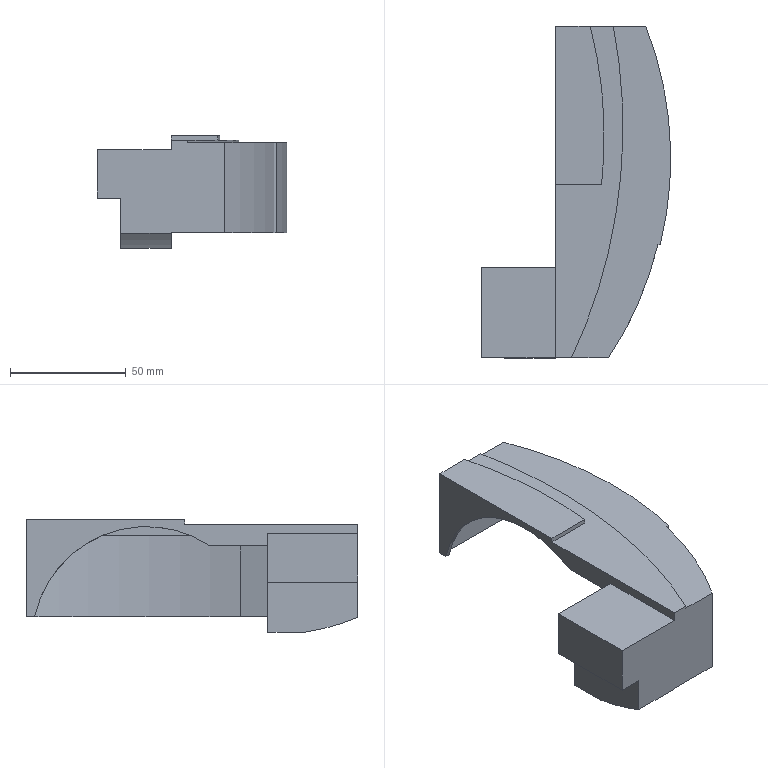Component | NX | WHEEL_MOUNT | 1 solid | 41 faces | volume 67381 mm3 | plane 29 | cylinder 12 | commonest cylinder face diameters 30 x3 316 x1 469.33 x1 386.311 x1 205.35 x1 314 x1 310.499 x1 311.501 x1